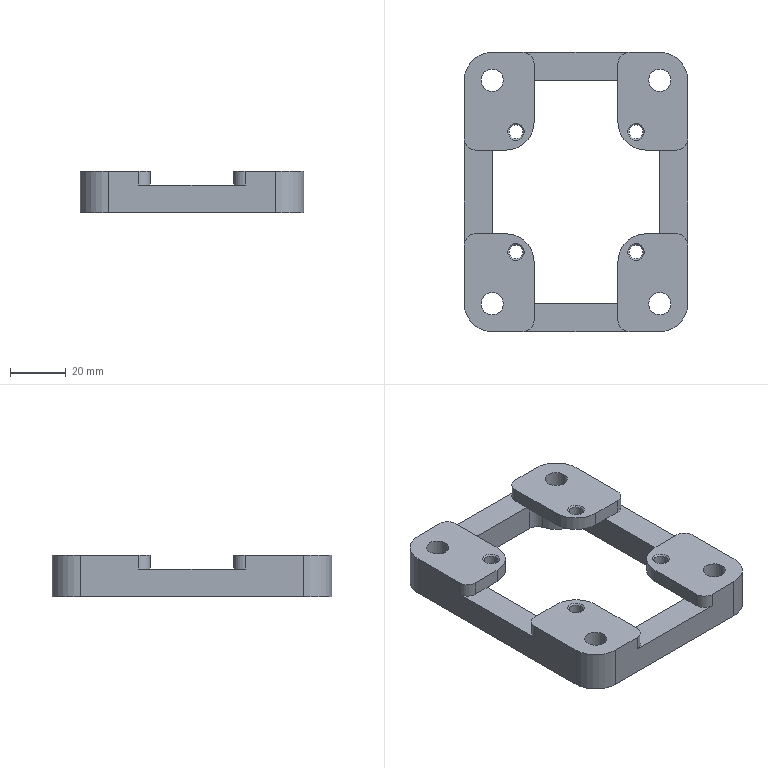Component | NX | CYLINDER_BASE | 1 solid | 73 faces | volume 47530 mm3 | cylinder 36 | plane 29 | cone 8 | commonest cylinder face diameters 8 x20 20 x12 5 x4